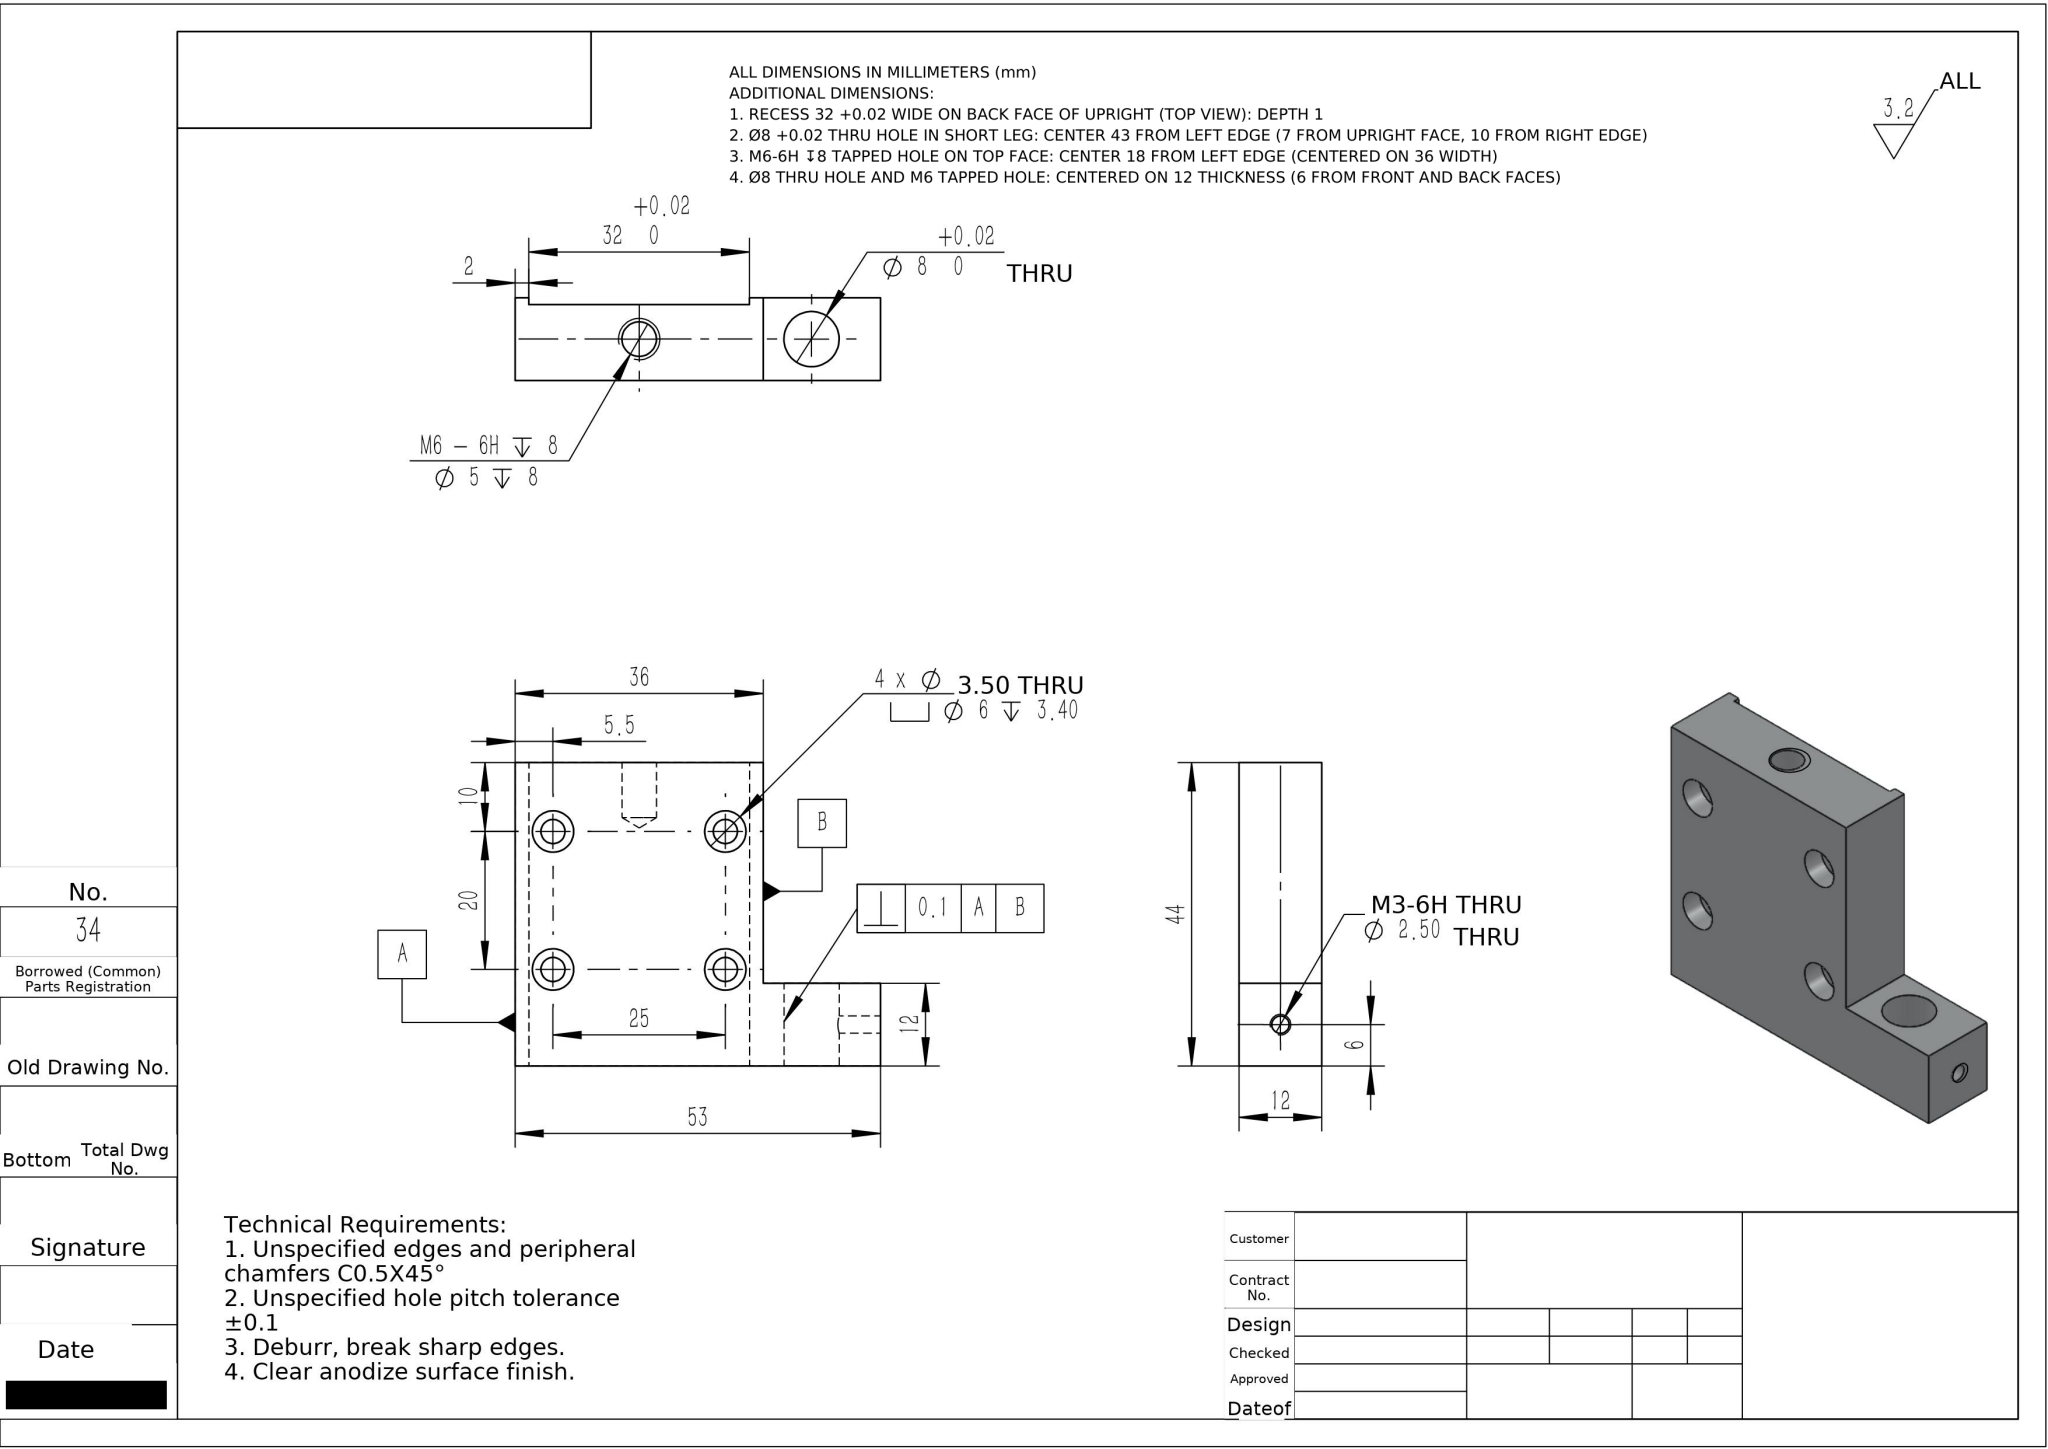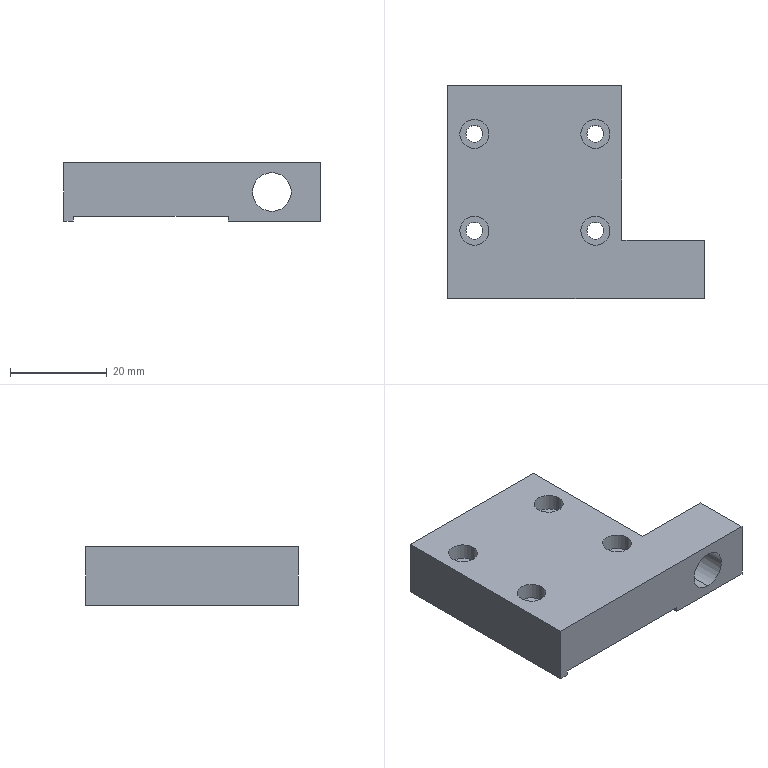Part | NX | mm | 1 solid | 40 faces | box 53 x 44 x 12 mm | volume 18571 mm3 | cylinder 22 | plane 16 | cone 2 | commonest cylinder face diameters 6 x8 3.5 x8 5 x2 2.5 x2 8 x2